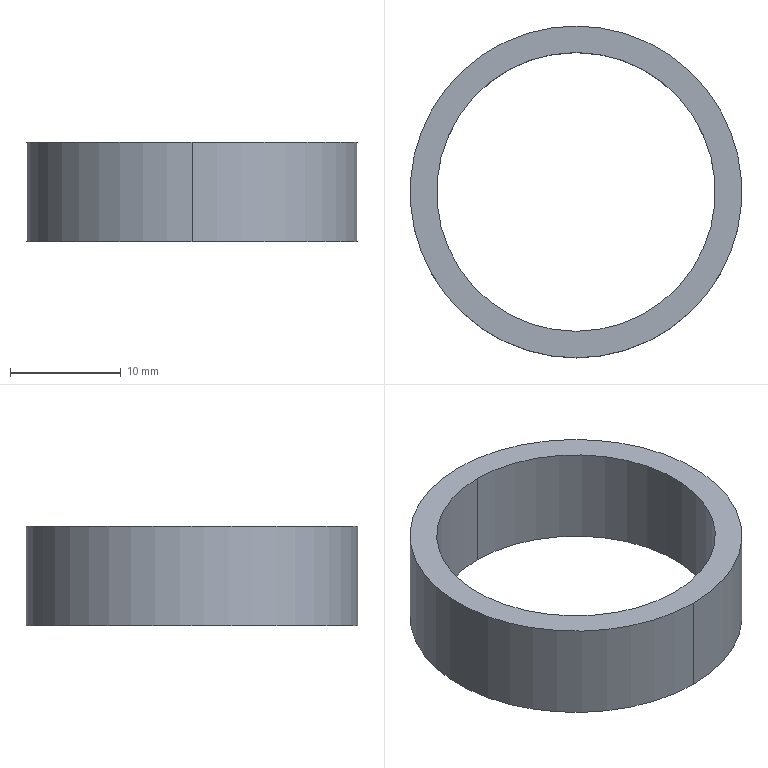Component | SolidWorks | TractionDriveWheelAssembly-1_TractionDriveWheelLimitSleeve2-1 | 1 solid | 6 faces | box 30 x 30 x 9 mm | volume 1873 mm3 | cylinder 4 | plane 2 | commonest cylinder face diameters 25.2 x2 30 x2
build123d program:
from build123d import *

# Parameters (mm, degrees)
SKETCH1_R           = 15
SKETCH1_R_2         = 12.6
BOSS_EXTRUDE1_DEPTH = 4.5


with BuildPart() as part:
    # Sketch1 → Boss-Extrude1 (new, symmetric)
    with BuildSketch(Plane.XY):
        Circle(SKETCH1_R)
        Circle(SKETCH1_R_2, mode=Mode.SUBTRACT)
    extrude(amount=BOSS_EXTRUDE1_DEPTH, both=True)


solid = part.part

# Placed as in the assembly
solid = solid.moved(Location((-299.507, -39.911, 619.5), (0, 0, 0)))
STEP:
#1=COLOUR_RGB('',0.7922,0.8196,0.9333);
#2=FILL_AREA_STYLE_COLOUR('',#1);
#3=FILL_AREA_STYLE('',(#2));
#4=SURFACE_STYLE_FILL_AREA(#3);
#5=SURFACE_SIDE_STYLE('',(#4));
#6=SURFACE_STYLE_USAGE(.BOTH.,#5);
#7=PRESENTATION_STYLE_ASSIGNMENT((#6));
#8=CARTESIAN_POINT('',(-11.792,-2.067,24.567));
#9=VERTEX_POINT('',#8);
#10=CARTESIAN_POINT('',(-11.792,-1.075,24.567));
#11=VERTEX_POINT('',#10);
#12=CARTESIAN_POINT('',(-11.792,-1.571,24.567));
#13=DIRECTION('',(-0.,-0.,1.));
#14=DIRECTION('',(-0.,1.,0.));
#15=AXIS2_PLACEMENT_3D('',#12,#13,#14);
#16=CIRCLE('',#15,0.4961);
#17=EDGE_CURVE('',#9,#11,#16,.T.);
#18=ORIENTED_EDGE('',*,*,#17,.T.);
#19=CARTESIAN_POINT('',(-11.792,-1.075,24.213));
#20=VERTEX_POINT('',#19);
#21=CARTESIAN_POINT('',(-11.792,-1.075,24.567));
#22=DIRECTION('',(0.,0.,-1.));
#23=VECTOR('',#22,39.37);
#24=LINE('',#21,#23);
#25=EDGE_CURVE('',#11,#20,#24,.T.);
#26=ORIENTED_EDGE('',*,*,#25,.T.);
#27=CARTESIAN_POINT('',(-11.792,-2.067,24.213));
#28=VERTEX_POINT('',#27);
#29=CARTESIAN_POINT('',(-11.792,-1.571,24.213));
#30=DIRECTION('',(-0.,-0.,1.));
#31=DIRECTION('',(-0.,1.,0.));
#32=AXIS2_PLACEMENT_3D('',#29,#30,#31);
#33=CIRCLE('',#32,0.4961);
#34=EDGE_CURVE('',#28,#20,#33,.T.);
#35=ORIENTED_EDGE('',*,*,#34,.F.);
#36=CARTESIAN_POINT('',(-11.792,-2.067,24.567));
#37=DIRECTION('',(0.,0.,-1.));
#38=VECTOR('',#37,39.37);
#39=LINE('',#36,#38);
#40=EDGE_CURVE('',#9,#28,#39,.T.);
#41=ORIENTED_EDGE('',*,*,#40,.F.);
#42=EDGE_LOOP('',(#18,#26,#35,#41));
#43=FACE_OUTER_BOUND('',#42,.T.);
#44=CARTESIAN_POINT('',(-11.792,-1.571,24.567));
#45=DIRECTION('',(0.,0.,-1.));
#46=DIRECTION('',(0.,-1.,0.));
#47=AXIS2_PLACEMENT_3D('',#44,#45,#46);
#48=CYLINDRICAL_SURFACE('',#47,0.4961);
#49=ADVANCED_FACE('',(#43),#48,.F.);
#50=CARTESIAN_POINT('',(-11.792,-0.9808,24.567));
#51=VERTEX_POINT('',#50);
#52=CARTESIAN_POINT('',(-11.792,-2.162,24.567));
#53=VERTEX_POINT('',#52);
#54=CARTESIAN_POINT('',(-11.792,-1.571,24.567));
#55=DIRECTION('',(-0.,-0.,1.));
#56=DIRECTION('',(-0.,1.,0.));
#57=AXIS2_PLACEMENT_3D('',#54,#55,#56);
#58=CIRCLE('',#57,0.5906);
#59=EDGE_CURVE('',#51,#53,#58,.T.);
#60=ORIENTED_EDGE('',*,*,#59,.F.);
#61=CARTESIAN_POINT('',(-11.792,-0.9808,24.213));
#62=VERTEX_POINT('',#61);
#63=CARTESIAN_POINT('',(-11.792,-0.9808,24.567));
#64=DIRECTION('',(0.,0.,-1.));
#65=VECTOR('',#64,39.37);
#66=LINE('',#63,#65);
#67=EDGE_CURVE('',#51,#62,#66,.T.);
#68=ORIENTED_EDGE('',*,*,#67,.T.);
#69=CARTESIAN_POINT('',(-11.792,-2.162,24.213));
#70=VERTEX_POINT('',#69);
#71=CARTESIAN_POINT('',(-11.792,-1.571,24.213));
#72=DIRECTION('',(-0.,-0.,1.));
#73=DIRECTION('',(-0.,1.,0.));
#74=AXIS2_PLACEMENT_3D('',#71,#72,#73);
#75=CIRCLE('',#74,0.5906);
#76=EDGE_CURVE('',#62,#70,#75,.T.);
#77=ORIENTED_EDGE('',*,*,#76,.T.);
#78=CARTESIAN_POINT('',(-11.792,-2.162,24.567));
#79=DIRECTION('',(0.,0.,-1.));
#80=VECTOR('',#79,39.37);
#81=LINE('',#78,#80);
#82=EDGE_CURVE('',#53,#70,#81,.T.);
#83=ORIENTED_EDGE('',*,*,#82,.F.);
#84=EDGE_LOOP('',(#60,#68,#77,#83));
#85=FACE_OUTER_BOUND('',#84,.T.);
#86=CARTESIAN_POINT('',(-11.792,-1.571,24.567));
#87=DIRECTION('',(0.,0.,-1.));
#88=DIRECTION('',(0.,-1.,0.));
#89=AXIS2_PLACEMENT_3D('',#86,#87,#88);
#90=CYLINDRICAL_SURFACE('',#89,0.5906);
#91=ADVANCED_FACE('',(#85),#90,.T.);
#92=CARTESIAN_POINT('',(-11.792,-1.571,24.567));
#93=DIRECTION('',(-0.,-0.,1.));
#94=DIRECTION('',(-0.,1.,0.));
#95=AXIS2_PLACEMENT_3D('',#92,#93,#94);
#96=CIRCLE('',#95,0.5906);
#97=EDGE_CURVE('',#53,#51,#96,.T.);
#98=ORIENTED_EDGE('',*,*,#97,.T.);
#99=ORIENTED_EDGE('',*,*,#59,.T.);
#100=EDGE_LOOP('',(#98,#99));
#101=FACE_OUTER_BOUND('',#100,.T.);
#102=ORIENTED_EDGE('',*,*,#17,.F.);
#103=CARTESIAN_POINT('',(-11.792,-1.571,24.567));
#104=DIRECTION('',(-0.,-0.,1.));
#105=DIRECTION('',(-0.,1.,0.));
#106=AXIS2_PLACEMENT_3D('',#103,#104,#105);
#107=CIRCLE('',#106,0.4961);
#108=EDGE_CURVE('',#11,#9,#107,.T.);
#109=ORIENTED_EDGE('',*,*,#108,.F.);
#110=EDGE_LOOP('',(#102,#109));
#111=FACE_BOUND('',#110,.T.);
#112=CARTESIAN_POINT('',(-11.792,-1.571,24.567));
#113=DIRECTION('',(-0.,-0.,1.));
#114=DIRECTION('',(-0.,1.,0.));
#115=AXIS2_PLACEMENT_3D('',#112,#113,#114);
#116=PLANE('',#115);
#117=ADVANCED_FACE('',(#101,#111),#116,.T.);
#118=CARTESIAN_POINT('',(-11.792,-1.571,24.213));
#119=DIRECTION('',(-0.,-0.,1.));
#120=DIRECTION('',(-0.,1.,0.));
#121=AXIS2_PLACEMENT_3D('',#118,#119,#120);
#122=CIRCLE('',#121,0.5906);
#123=EDGE_CURVE('',#70,#62,#122,.T.);
#124=ORIENTED_EDGE('',*,*,#123,.F.);
#125=ORIENTED_EDGE('',*,*,#76,.F.);
#126=EDGE_LOOP('',(#124,#125));
#127=FACE_OUTER_BOUND('',#126,.T.);
#128=ORIENTED_EDGE('',*,*,#34,.T.);
#129=CARTESIAN_POINT('',(-11.792,-1.571,24.213));
#130=DIRECTION('',(-0.,-0.,1.));
#131=DIRECTION('',(-0.,1.,0.));
#132=AXIS2_PLACEMENT_3D('',#129,#130,#131);
#133=CIRCLE('',#132,0.4961);
#134=EDGE_CURVE('',#20,#28,#133,.T.);
#135=ORIENTED_EDGE('',*,*,#134,.T.);
#136=EDGE_LOOP('',(#128,#135));
#137=FACE_BOUND('',#136,.T.);
#138=CARTESIAN_POINT('',(-11.792,-1.571,24.213));
#139=DIRECTION('',(-0.,-0.,1.));
#140=DIRECTION('',(-0.,1.,0.));
#141=AXIS2_PLACEMENT_3D('',#138,#139,#140);
#142=PLANE('',#141);
#143=ADVANCED_FACE('',(#127,#137),#142,.F.);
#144=ORIENTED_EDGE('',*,*,#67,.F.);
#145=ORIENTED_EDGE('',*,*,#97,.F.);
#146=ORIENTED_EDGE('',*,*,#82,.T.);
#147=ORIENTED_EDGE('',*,*,#123,.T.);
#148=EDGE_LOOP('',(#144,#145,#146,#147));
#149=FACE_OUTER_BOUND('',#148,.T.);
#150=CARTESIAN_POINT('',(-11.792,-1.571,24.567));
#151=DIRECTION('',(0.,0.,-1.));
#152=DIRECTION('',(0.,-1.,0.));
#153=AXIS2_PLACEMENT_3D('',#150,#151,#152);
#154=CYLINDRICAL_SURFACE('',#153,0.5906);
#155=ADVANCED_FACE('',(#149),#154,.T.);
#156=ORIENTED_EDGE('',*,*,#25,.F.);
#157=ORIENTED_EDGE('',*,*,#108,.T.);
#158=ORIENTED_EDGE('',*,*,#40,.T.);
#159=ORIENTED_EDGE('',*,*,#134,.F.);
#160=EDGE_LOOP('',(#156,#157,#158,#159));
#161=FACE_OUTER_BOUND('',#160,.T.);
#162=CARTESIAN_POINT('',(-11.792,-1.571,24.567));
#163=DIRECTION('',(0.,0.,-1.));
#164=DIRECTION('',(0.,-1.,0.));
#165=AXIS2_PLACEMENT_3D('',#162,#163,#164);
#166=CYLINDRICAL_SURFACE('',#165,0.4961);
#167=ADVANCED_FACE('',(#161),#166,.F.);
#168=CLOSED_SHELL('',(#49,#91,#117,#143,#155,#167));
#169=MANIFOLD_SOLID_BREP('',#168);
#170=STYLED_ITEM('',(#7),#169);
#171=PRESENTATION_LAYER_ASSIGNMENT('','',(#170));
#172=(LENGTH_UNIT()NAMED_UNIT(*)SI_UNIT($,.METRE.));
#173=LENGTH_MEASURE_WITH_UNIT(LENGTH_MEASURE(0.0254),#172);
#174=DIMENSIONAL_EXPONENTS(1.,0.,0.,0.,0.,0.,0.);
#175=(CONVERSION_BASED_UNIT('',#173)LENGTH_UNIT()NAMED_UNIT(#174));
#176=UNCERTAINTY_MEASURE_WITH_UNIT(LENGTH_MEASURE(0.00001),#175,'','');
#177=(NAMED_UNIT(*)PLANE_ANGLE_UNIT()SI_UNIT($,.RADIAN.));
#178=(NAMED_UNIT(*)SI_UNIT($,.STERADIAN.)SOLID_ANGLE_UNIT());
#179=(GEOMETRIC_REPRESENTATION_CONTEXT(3)GLOBAL_UNCERTAINTY_ASSIGNED_CONTEXT((#176))GLOBAL_UNIT_ASSIGNED_CONTEXT((#175,#177,#178))REPRESENTATION_CONTEXT('',''));
#180=MECHANICAL_DESIGN_GEOMETRIC_PRESENTATION_REPRESENTATION('',(#170),#179);
#181=CARTESIAN_POINT('',(0.,0.,0.));
#182=DIRECTION('',(0.,0.,1.));
#183=DIRECTION('',(1.,0.,0.));
#184=AXIS2_PLACEMENT_3D('',#181,#182,#183);
#185=(LENGTH_UNIT()NAMED_UNIT(*)SI_UNIT($,.METRE.));
#186=LENGTH_MEASURE_WITH_UNIT(LENGTH_MEASURE(0.0254),#185);
#187=DIMENSIONAL_EXPONENTS(1.,0.,0.,0.,0.,0.,0.);
#188=(CONVERSION_BASED_UNIT('',#186)LENGTH_UNIT()NAMED_UNIT(#187));
#189=UNCERTAINTY_MEASURE_WITH_UNIT(LENGTH_MEASURE(0.00001),#188,'','');
#190=(NAMED_UNIT(*)PLANE_ANGLE_UNIT()SI_UNIT($,.RADIAN.));
#191=(NAMED_UNIT(*)SI_UNIT($,.STERADIAN.)SOLID_ANGLE_UNIT());
#192=(GEOMETRIC_REPRESENTATION_CONTEXT(3)GLOBAL_UNCERTAINTY_ASSIGNED_CONTEXT((#189))GLOBAL_UNIT_ASSIGNED_CONTEXT((#188,#190,#191))REPRESENTATION_CONTEXT('',''));
#193=ADVANCED_BREP_SHAPE_REPRESENTATION('',(#169,#184),#192);